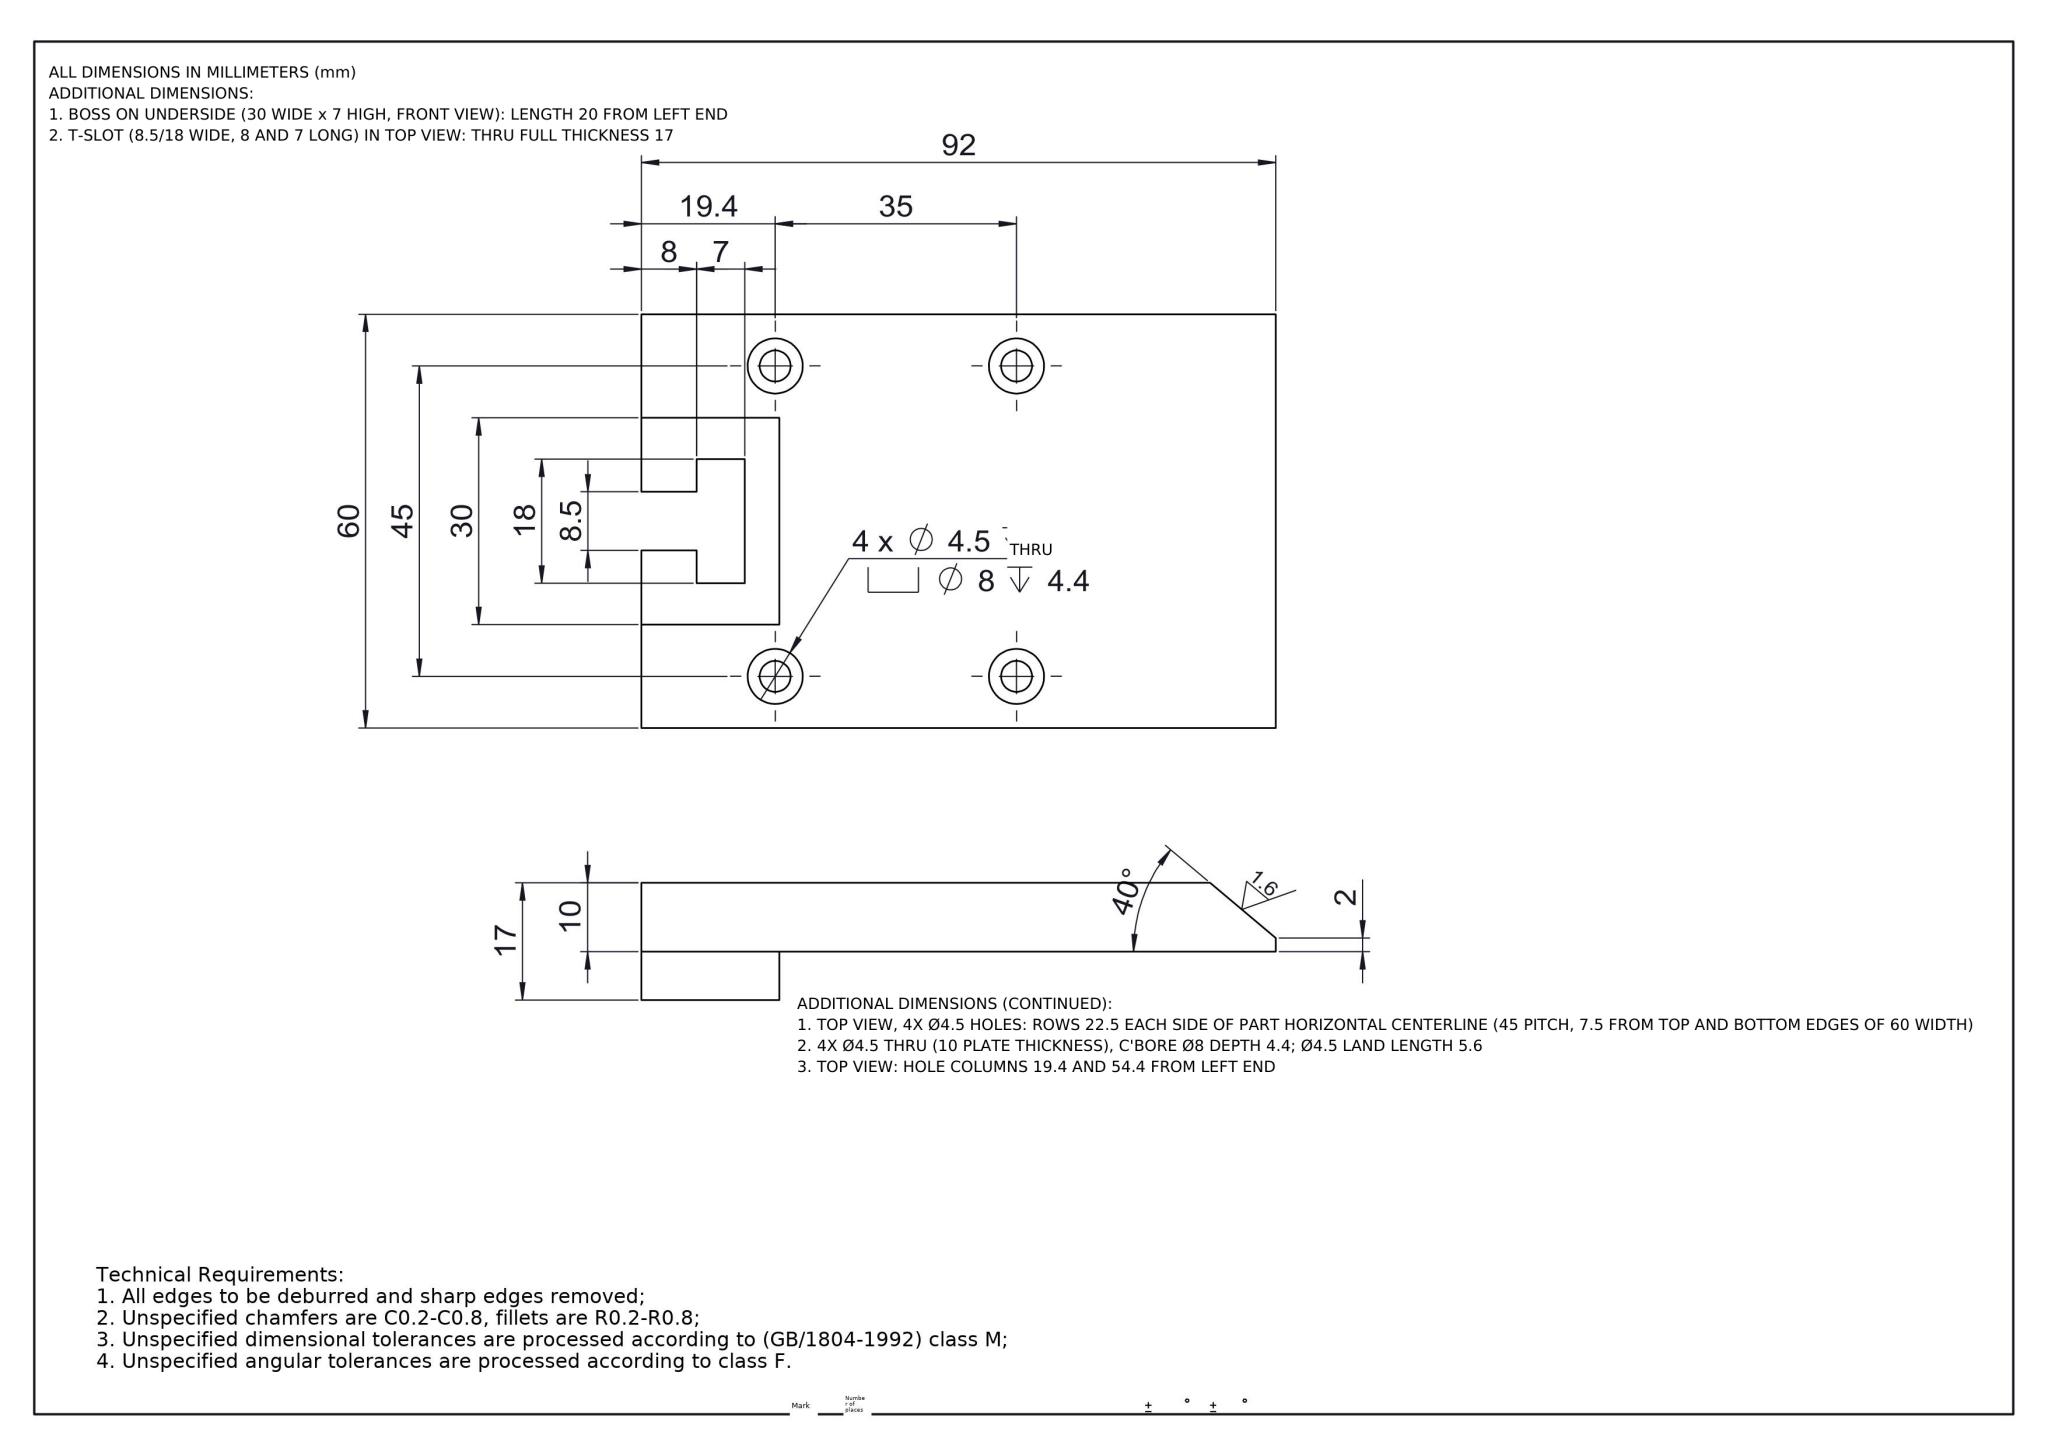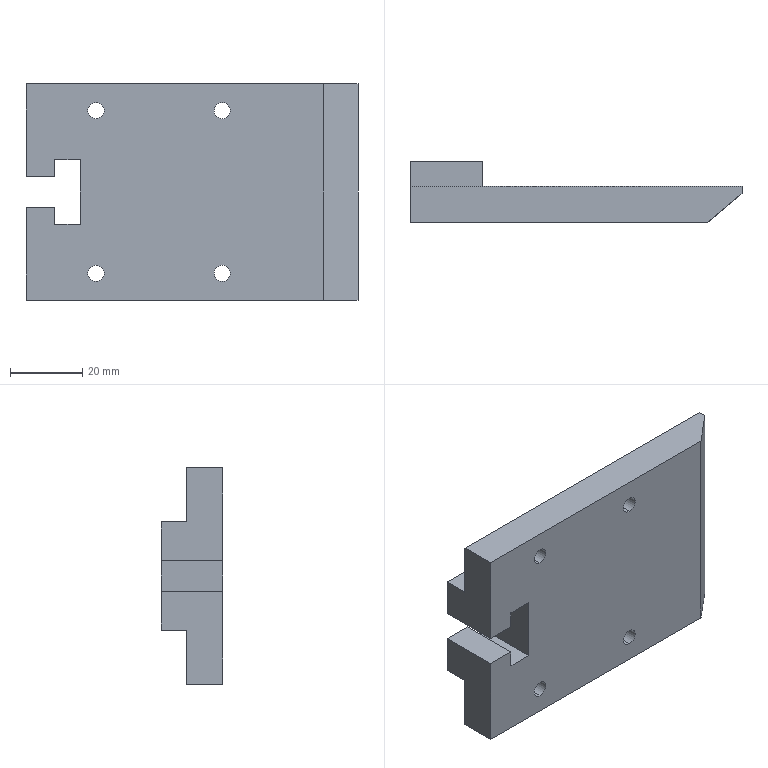Part | NX | mm | 1 solid | 39 faces | box 92 x 17 x 60 mm | volume 52573 mm3 | plane 23 | cylinder 16 | commonest cylinder face diameters 8 x8 4.5 x8